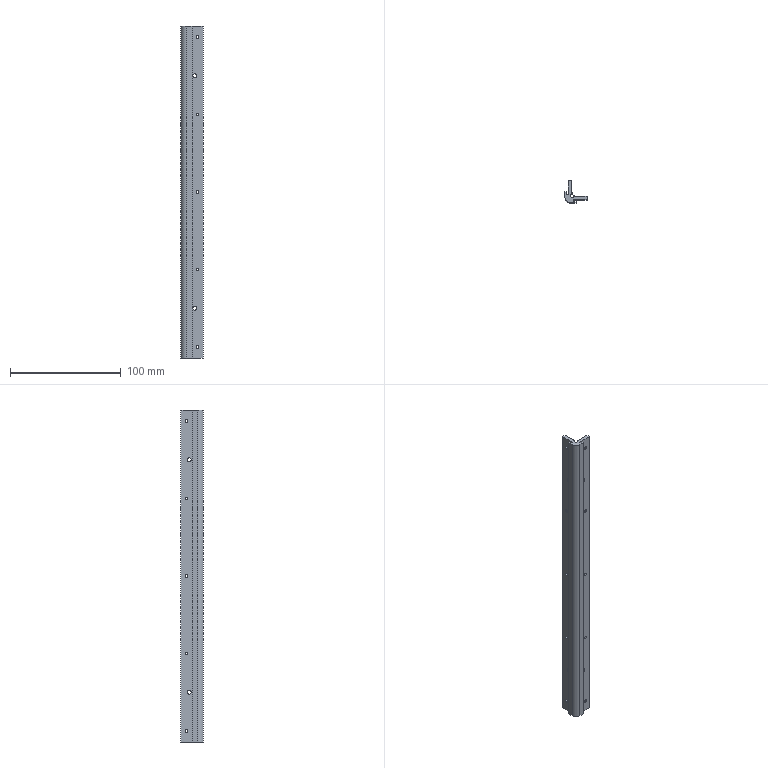CAM job | Mastercam | mm | 4 operations | part box 20 x 20 x 300
1. Contour (Ramp) | 8 - 8 平铣刀
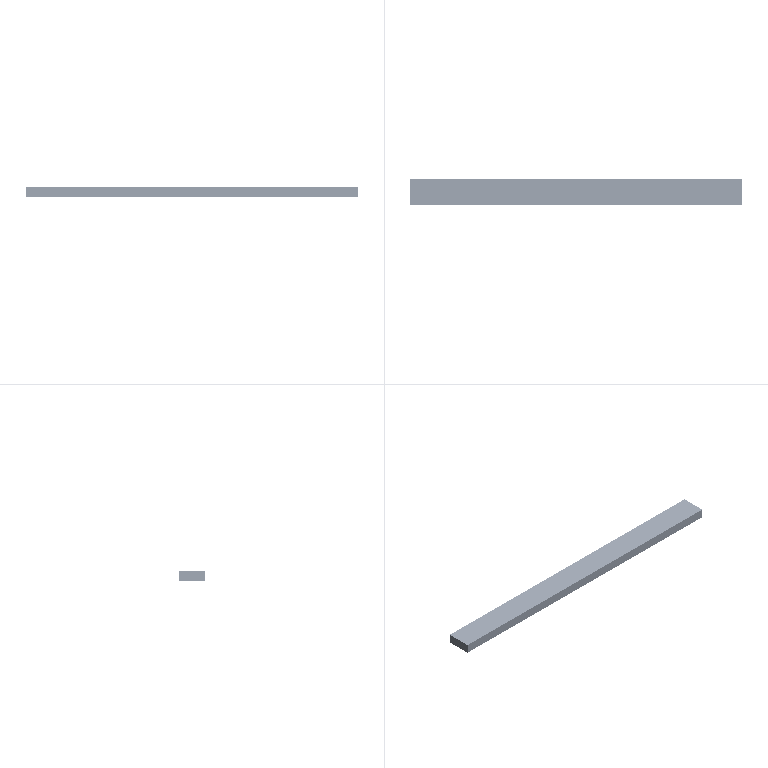2. Contour (2D) | 8 - 8 平铣刀
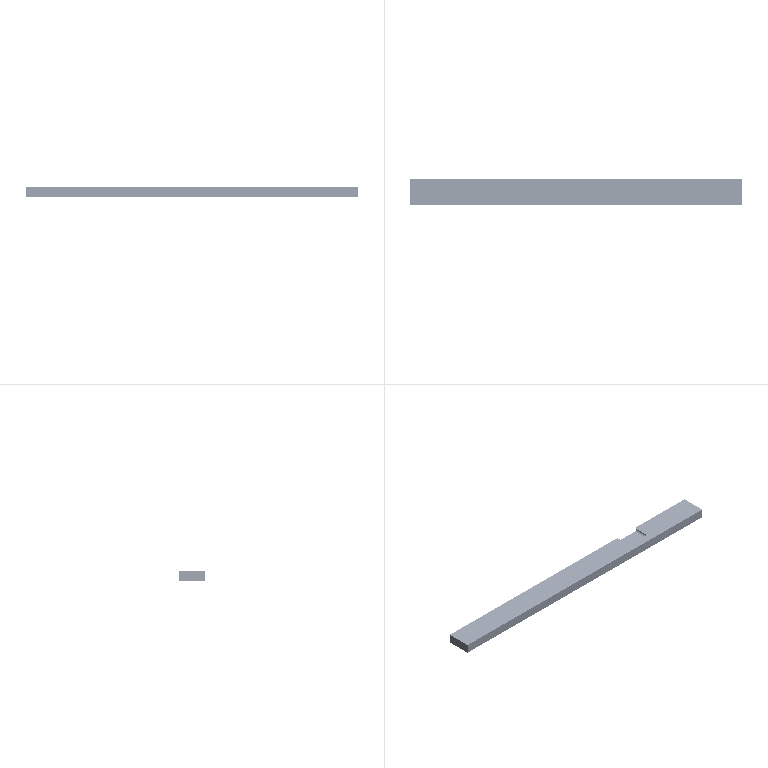3. Drill/Counterbore | 7 - 4 倒角刀
4. Drill/Counterbore | 7 - 4 倒角刀